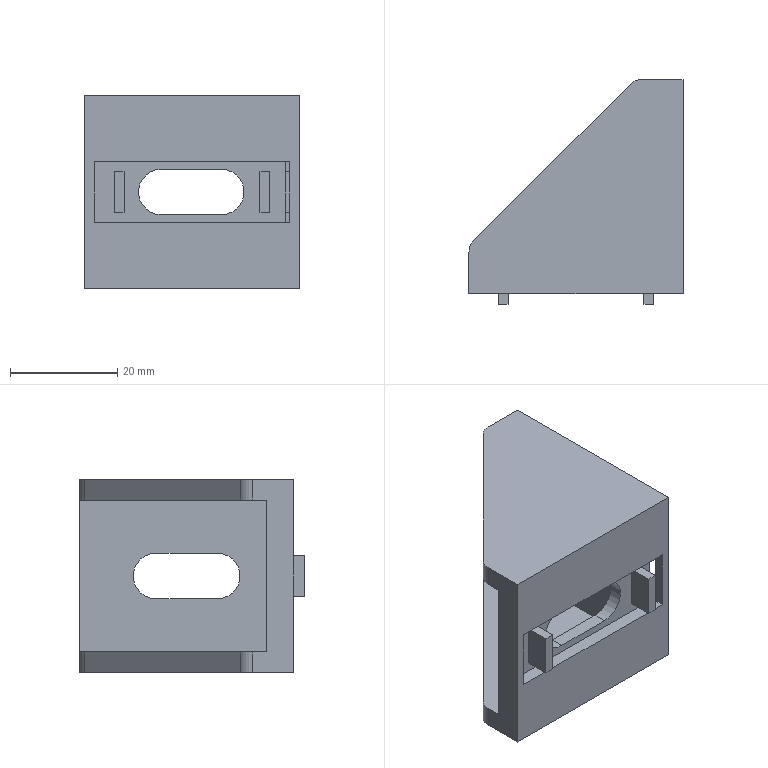Component | SolidWorks | NewG408-4040NationalStandardAngleCode-2 | 1 solid | 52 faces | volume 16506 mm3 | plane 44 | cylinder 8 | commonest cylinder face diameters 6 x4 8.5 x4 | material A6061